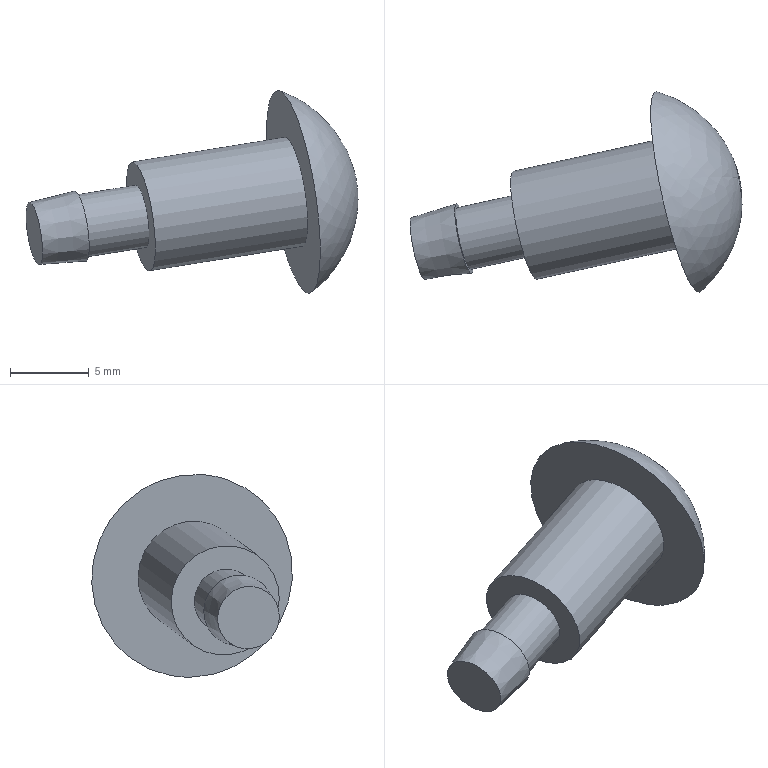Component | NX | 2_13 | 1 solid | 8 faces | box 21.02 x 12.71 x 12.84 mm | volume 772 mm3 | plane 4 | cylinder 2 | spline 1 | cone 1 | commonest cylinder face diameters 7 x1 4 x1
STEP:
#1=CARTESIAN_POINT('',(0.,0.,0.));
#2=DIRECTION('',(0.,0.,1.));
#3=DIRECTION('',(1.,0.,0.));
#4=AXIS2_PLACEMENT_3D('',#1,#2,#3);
#5=CARTESIAN_POINT('',(138.921,125.393,-187.423));
#6=VERTEX_POINT('',#5);
#7=CARTESIAN_POINT('',(139.276,125.209,-189.382));
#8=DIRECTION('',(0.9653,0.21,0.1554));
#9=DIRECTION('',(-0.1779,0.09244,0.9797));
#10=AXIS2_PLACEMENT_3D('',#7,#8,#9);
#11=CIRCLE('',#10,2.);
#12=CARTESIAN_POINT('',(139.632,125.024,-191.342));
#13=DIRECTION('',(-0.9653,-0.21,-0.1554));
#14=DIRECTION('',(0.1779,-0.09244,-0.9797));
#15=AXIS2_PLACEMENT_3D('',#12,#13,#14);
#16=PLANE('',#15);
#17=CARTESIAN_POINT('',(-4.,0.));
#18=CARTESIAN_POINT('',(-4.,3.464));
#19=CARTESIAN_POINT('',(-1.,1.732));
#20=CARTESIAN_POINT('',(2.,0.));
#21=CARTESIAN_POINT('',(-1.,-1.732));
#22=CARTESIAN_POINT('',(-4.,-3.464));
#23=CARTESIAN_POINT('',(-4.,0.));
#24=(BOUNDED_CURVE()B_SPLINE_CURVE(2,(#17,#18,#19,#20,#21,#22,#23),.UNSPECIFIED.,.T.,.F.)B_SPLINE_CURVE_WITH_KNOTS((1,2,2,2,2,1),(-2.094,0.,2.094,4.189,6.283,8.378),.UNSPECIFIED.)CURVE()GEOMETRIC_REPRESENTATION_ITEM()RATIONAL_B_SPLINE_CURVE((1.,0.5,1.,0.5,1.,0.5,1.))REPRESENTATION_ITEM(''));
#25=(GEOMETRIC_REPRESENTATION_CONTEXT(2)PARAMETRIC_REPRESENTATION_CONTEXT()REPRESENTATION_CONTEXT('',''));
#26=DEFINITIONAL_REPRESENTATION('',(#24),#25);
#27=PCURVE('',#16,#26);
#28=CARTESIAN_POINT('',(142.172,125.839,-188.916));
#29=DIRECTION('',(0.9653,0.21,0.1554));
#30=DIRECTION('',(-0.1779,0.09244,0.9797));
#31=AXIS2_PLACEMENT_3D('',#28,#29,#30);
#32=CONICAL_SURFACE('',#31,2.25,0.08314);
#33=CARTESIAN_POINT('',(0.,-3.));
#34=DIRECTION('',(1.,0.));
#35=VECTOR('',#34,1.);
#36=LINE('',#33,#35);
#37=(GEOMETRIC_REPRESENTATION_CONTEXT(2)PARAMETRIC_REPRESENTATION_CONTEXT()REPRESENTATION_CONTEXT('',''));
#38=DEFINITIONAL_REPRESENTATION('',(#36),#37);
#39=PCURVE('',#32,#38);
#40=SURFACE_CURVE('',#11,(#27,#39),.PCURVE_S1.);
#41=EDGE_CURVE('',#6,#6,#40,.T.);
#42=ORIENTED_EDGE('',*,*,#41,.F.);
#43=EDGE_LOOP('',(#42));
#44=FACE_BOUND('',#43,.T.);
#45=ADVANCED_FACE('',(#44),#16,.T.);
#46=CARTESIAN_POINT('',(154.53,129.379,-180.372));
#47=VERTEX_POINT('',#46);
#48=CARTESIAN_POINT('',(155.686,128.779,-186.74));
#49=DIRECTION('',(0.9653,0.21,0.1554));
#50=DIRECTION('',(-0.1779,0.09244,0.9797));
#51=AXIS2_PLACEMENT_3D('',#48,#49,#50);
#52=CIRCLE('',#51,6.5);
#53=CARTESIAN_POINT('',(159.547,129.619,-186.118));
#54=CARTESIAN_POINT('',(159.547,129.619,-186.118));
#55=CARTESIAN_POINT('',(159.547,129.619,-186.118));
#56=CARTESIAN_POINT('',(159.547,129.619,-186.118));
#57=CARTESIAN_POINT('',(159.547,129.619,-186.118));
#58=CARTESIAN_POINT('',(159.547,129.619,-186.118));
#59=CARTESIAN_POINT('',(159.547,129.619,-186.118));
#60=CARTESIAN_POINT('',(159.,129.867,-183.379));
#61=CARTESIAN_POINT('',(160.073,124.409,-182.669));
#62=CARTESIAN_POINT('',(161.07,123.891,-188.163));
#63=CARTESIAN_POINT('',(159.997,129.349,-188.873));
#64=CARTESIAN_POINT('',(158.924,134.807,-189.582));
#65=CARTESIAN_POINT('',(157.927,135.325,-184.089));
#66=CARTESIAN_POINT('',(159.,129.867,-183.379));
#67=CARTESIAN_POINT('',(157.157,129.779,-181.268));
#68=CARTESIAN_POINT('',(159.144,119.673,-179.953));
#69=CARTESIAN_POINT('',(160.991,118.713,-190.126));
#70=CARTESIAN_POINT('',(159.003,128.82,-191.441));
#71=CARTESIAN_POINT('',(157.016,138.926,-192.755));
#72=CARTESIAN_POINT('',(155.169,139.886,-182.582));
#73=CARTESIAN_POINT('',(157.157,129.779,-181.268));
#74=CARTESIAN_POINT('',(154.53,129.379,-180.372));
#75=CARTESIAN_POINT('',(157.018,116.726,-178.726));
#76=CARTESIAN_POINT('',(159.33,115.525,-191.462));
#77=CARTESIAN_POINT('',(156.842,128.178,-193.108));
#78=CARTESIAN_POINT('',(154.354,140.831,-194.753));
#79=CARTESIAN_POINT('',(152.042,142.033,-182.017));
#80=CARTESIAN_POINT('',(154.53,129.379,-180.372));
#81=(BOUNDED_SURFACE()B_SPLINE_SURFACE(3,3,((#53,#54,#55,#56,#57,#58,#59),(#60,#61,#62,#63,#64,#65,#66),(#67,#68,#69,#70,#71,#72,#73),(#74,#75,#76,#77,#78,#79,#80)),.UNSPECIFIED.,.F.,.T.,.F.)B_SPLINE_SURFACE_WITH_KNOTS((4,4),(1,3,3,3,1),(0.,1.),(-0.5,0.,0.5,1.,1.5),.UNSPECIFIED.)GEOMETRIC_REPRESENTATION_ITEM()RATIONAL_B_SPLINE_SURFACE(((1.,0.3333,0.3333,1.,0.3333,0.3333,1.),(0.9073,0.3024,0.3024,0.9073,0.3024,0.3024,0.9073),(0.9073,0.3024,0.3024,0.9073,0.3024,0.3024,0.9073),(1.,0.3333,0.3333,1.,0.3333,0.3333,1.)))REPRESENTATION_ITEM('')SURFACE());
#82=CARTESIAN_POINT('',(1.,0.));
#83=CARTESIAN_POINT('',(1.,0.02352));
#84=CARTESIAN_POINT('',(1.,0.06491));
#85=CARTESIAN_POINT('',(1.,0.1146));
#86=CARTESIAN_POINT('',(1.,0.1575));
#87=CARTESIAN_POINT('',(1.,0.196));
#88=CARTESIAN_POINT('',(1.,0.2322));
#89=CARTESIAN_POINT('',(1.,0.2678));
#90=CARTESIAN_POINT('',(1.,0.304));
#91=CARTESIAN_POINT('',(1.,0.3425));
#92=CARTESIAN_POINT('',(1.,0.3856));
#93=CARTESIAN_POINT('',(1.,0.4343));
#94=CARTESIAN_POINT('',(1.,0.5));
#95=CARTESIAN_POINT('',(1.,0.5657));
#96=CARTESIAN_POINT('',(1.,0.6144));
#97=CARTESIAN_POINT('',(1.,0.6575));
#98=CARTESIAN_POINT('',(1.,0.696));
#99=CARTESIAN_POINT('',(1.,0.7322));
#100=CARTESIAN_POINT('',(1.,0.7678));
#101=CARTESIAN_POINT('',(1.,0.804));
#102=CARTESIAN_POINT('',(1.,0.8425));
#103=CARTESIAN_POINT('',(1.,0.8854));
#104=CARTESIAN_POINT('',(1.,0.9351));
#105=CARTESIAN_POINT('',(1.,0.9765));
#106=CARTESIAN_POINT('',(1.,1.));
#107=B_SPLINE_CURVE_WITH_KNOTS('',3,(#82,#83,#84,#85,#86,#87,#88,#89,#90,#91,#92,#93,#94,#95,#96,#97,#98,#99,#100,#101,#102,#103,#104,#105,#106),.UNSPECIFIED.,.F.,.F.,(4,1,1,1,1,1,1,1,1,1,1,1,1,1,1,1,1,1,1,1,1,1,4),(0.,0.2856,0.5712,0.8568,1.142,1.428,1.714,1.999,2.285,2.57,2.856,3.142,3.427,3.713,3.998,4.284,4.57,4.855,5.141,5.426,5.712,5.998,6.283),.QUASI_UNIFORM_KNOTS.);
#108=(GEOMETRIC_REPRESENTATION_CONTEXT(2)PARAMETRIC_REPRESENTATION_CONTEXT()REPRESENTATION_CONTEXT('',''));
#109=DEFINITIONAL_REPRESENTATION('',(#107),#108);
#110=PCURVE('',#81,#109);
#111=CARTESIAN_POINT('',(156.842,128.178,-193.108));
#112=DIRECTION('',(-0.9653,-0.21,-0.1554));
#113=DIRECTION('',(0.1779,-0.09244,-0.9797));
#114=AXIS2_PLACEMENT_3D('',#111,#112,#113);
#115=PLANE('',#114);
#116=CARTESIAN_POINT('',(-13.,-0.));
#117=CARTESIAN_POINT('',(-13.,11.258));
#118=CARTESIAN_POINT('',(-3.25,5.629));
#119=CARTESIAN_POINT('',(6.5,-0.));
#120=CARTESIAN_POINT('',(-3.25,-5.629));
#121=CARTESIAN_POINT('',(-13.,-11.258));
#122=CARTESIAN_POINT('',(-13.,-0.));
#123=(BOUNDED_CURVE()B_SPLINE_CURVE(2,(#116,#117,#118,#119,#120,#121,#122),.UNSPECIFIED.,.T.,.F.)B_SPLINE_CURVE_WITH_KNOTS((1,2,2,2,2,1),(-2.094,0.,2.094,4.189,6.283,8.378),.UNSPECIFIED.)CURVE()GEOMETRIC_REPRESENTATION_ITEM()RATIONAL_B_SPLINE_CURVE((1.,0.5,1.,0.5,1.,0.5,1.))REPRESENTATION_ITEM(''));
#124=(GEOMETRIC_REPRESENTATION_CONTEXT(2)PARAMETRIC_REPRESENTATION_CONTEXT()REPRESENTATION_CONTEXT('',''));
#125=DEFINITIONAL_REPRESENTATION('',(#123),#124);
#126=PCURVE('',#115,#125);
#127=SURFACE_CURVE('',#52,(#110,#126),.PCURVE_S1.);
#128=EDGE_CURVE('',#47,#47,#127,.T.);
#129=ORIENTED_EDGE('',*,*,#128,.T.);
#130=CARTESIAN_POINT('',(159.547,129.619,-186.118));
#131=VERTEX_POINT('',#130);
#132=CARTESIAN_POINT('',(159.547,129.619,-186.118));
#133=CARTESIAN_POINT('',(159.,129.867,-183.379));
#134=CARTESIAN_POINT('',(157.157,129.779,-181.268));
#135=CARTESIAN_POINT('',(154.53,129.379,-180.372));
#136=(BOUNDED_CURVE()B_SPLINE_CURVE(3,(#132,#133,#134,#135),.UNSPECIFIED.,.F.,.F.)B_SPLINE_CURVE_WITH_KNOTS((4,4),(0.,1.),.PIECEWISE_BEZIER_KNOTS.)CURVE()GEOMETRIC_REPRESENTATION_ITEM()RATIONAL_B_SPLINE_CURVE((1.,0.9073,0.9073,1.))REPRESENTATION_ITEM(''));
#137=CARTESIAN_POINT('',(0.,1.));
#138=DIRECTION('',(1.,0.));
#139=VECTOR('',#138,1.);
#140=LINE('',#137,#139);
#141=(GEOMETRIC_REPRESENTATION_CONTEXT(2)PARAMETRIC_REPRESENTATION_CONTEXT()REPRESENTATION_CONTEXT('',''));
#142=DEFINITIONAL_REPRESENTATION('',(#140),#141);
#143=PCURVE('',#81,#142);
#144=CARTESIAN_POINT('',(0.,0.));
#145=DIRECTION('',(1.,0.));
#146=VECTOR('',#145,1.);
#147=LINE('',#144,#146);
#148=(GEOMETRIC_REPRESENTATION_CONTEXT(2)PARAMETRIC_REPRESENTATION_CONTEXT()REPRESENTATION_CONTEXT('',''));
#149=DEFINITIONAL_REPRESENTATION('',(#147),#148);
#150=PCURVE('',#81,#149);
#151=SEAM_CURVE('',#136,(#143,#150),.PCURVE_S1.);
#152=EDGE_CURVE('',#131,#47,#151,.T.);
#153=ORIENTED_EDGE('',*,*,#152,.F.);
#154=ORIENTED_EDGE('',*,*,#152,.T.);
#155=EDGE_LOOP('',(#129,#153,#154));
#156=FACE_BOUND('',#155,.T.);
#157=ADVANCED_FACE('',(#156),#81,.T.);
#158=CARTESIAN_POINT('',(155.063,129.102,-183.311));
#159=VERTEX_POINT('',#158);
#160=CARTESIAN_POINT('',(155.686,128.779,-186.74));
#161=DIRECTION('',(0.9653,0.21,0.1554));
#162=DIRECTION('',(-0.1779,0.09244,0.9797));
#163=AXIS2_PLACEMENT_3D('',#160,#161,#162);
#164=CIRCLE('',#163,3.5);
#165=CARTESIAN_POINT('',(-10.,-0.));
#166=CARTESIAN_POINT('',(-10.,6.062));
#167=CARTESIAN_POINT('',(-4.75,3.031));
#168=CARTESIAN_POINT('',(0.5,-0.));
#169=CARTESIAN_POINT('',(-4.75,-3.031));
#170=CARTESIAN_POINT('',(-10.,-6.062));
#171=CARTESIAN_POINT('',(-10.,-0.));
#172=(BOUNDED_CURVE()B_SPLINE_CURVE(2,(#165,#166,#167,#168,#169,#170,#171),.UNSPECIFIED.,.T.,.F.)B_SPLINE_CURVE_WITH_KNOTS((1,2,2,2,2,1),(-2.094,0.,2.094,4.189,6.283,8.378),.UNSPECIFIED.)CURVE()GEOMETRIC_REPRESENTATION_ITEM()RATIONAL_B_SPLINE_CURVE((1.,0.5,1.,0.5,1.,0.5,1.))REPRESENTATION_ITEM(''));
#173=(GEOMETRIC_REPRESENTATION_CONTEXT(2)PARAMETRIC_REPRESENTATION_CONTEXT()REPRESENTATION_CONTEXT('',''));
#174=DEFINITIONAL_REPRESENTATION('',(#172),#173);
#175=PCURVE('',#115,#174);
#176=CARTESIAN_POINT('',(148.929,127.309,-187.828));
#177=DIRECTION('',(0.9653,0.21,0.1554));
#178=DIRECTION('',(-0.1779,0.09244,0.9797));
#179=AXIS2_PLACEMENT_3D('',#176,#177,#178);
#180=CYLINDRICAL_SURFACE('',#179,3.5);
#181=CARTESIAN_POINT('',(0.,7.));
#182=DIRECTION('',(1.,0.));
#183=VECTOR('',#182,1.);
#184=LINE('',#181,#183);
#185=(GEOMETRIC_REPRESENTATION_CONTEXT(2)PARAMETRIC_REPRESENTATION_CONTEXT()REPRESENTATION_CONTEXT('',''));
#186=DEFINITIONAL_REPRESENTATION('',(#184),#185);
#187=PCURVE('',#180,#186);
#188=SURFACE_CURVE('',#164,(#175,#187),.PCURVE_S1.);
#189=EDGE_CURVE('',#159,#159,#188,.T.);
#190=ORIENTED_EDGE('',*,*,#189,.T.);
#191=EDGE_LOOP('',(#190));
#192=FACE_BOUND('',#191,.T.);
#193=ORIENTED_EDGE('',*,*,#128,.F.);
#194=EDGE_LOOP('',(#193));
#195=FACE_BOUND('',#194,.T.);
#196=ADVANCED_FACE('',(#192,#195),#115,.T.);
#197=CARTESIAN_POINT('',(145.411,127.002,-184.865));
#198=VERTEX_POINT('',#197);
#199=CARTESIAN_POINT('',(146.033,126.679,-188.294));
#200=DIRECTION('',(0.9653,0.21,0.1554));
#201=DIRECTION('',(-0.1779,0.09244,0.9797));
#202=AXIS2_PLACEMENT_3D('',#199,#200,#201);
#203=CIRCLE('',#202,3.5);
#204=CARTESIAN_POINT('',(0.,-3.));
#205=DIRECTION('',(1.,0.));
#206=VECTOR('',#205,1.);
#207=LINE('',#204,#206);
#208=(GEOMETRIC_REPRESENTATION_CONTEXT(2)PARAMETRIC_REPRESENTATION_CONTEXT()REPRESENTATION_CONTEXT('',''));
#209=DEFINITIONAL_REPRESENTATION('',(#207),#208);
#210=PCURVE('',#180,#209);
#211=CARTESIAN_POINT('',(146.656,126.355,-191.723));
#212=DIRECTION('',(-0.9653,-0.21,-0.1554));
#213=DIRECTION('',(0.1779,-0.09244,-0.9797));
#214=AXIS2_PLACEMENT_3D('',#211,#212,#213);
#215=PLANE('',#214);
#216=CARTESIAN_POINT('',(-7.,-0.));
#217=CARTESIAN_POINT('',(-7.,6.062));
#218=CARTESIAN_POINT('',(-1.75,3.031));
#219=CARTESIAN_POINT('',(3.5,-0.));
#220=CARTESIAN_POINT('',(-1.75,-3.031));
#221=CARTESIAN_POINT('',(-7.,-6.062));
#222=CARTESIAN_POINT('',(-7.,-0.));
#223=(BOUNDED_CURVE()B_SPLINE_CURVE(2,(#216,#217,#218,#219,#220,#221,#222),.UNSPECIFIED.,.T.,.F.)B_SPLINE_CURVE_WITH_KNOTS((1,2,2,2,2,1),(-2.094,0.,2.094,4.189,6.283,8.378),.UNSPECIFIED.)CURVE()GEOMETRIC_REPRESENTATION_ITEM()RATIONAL_B_SPLINE_CURVE((1.,0.5,1.,0.5,1.,0.5,1.))REPRESENTATION_ITEM(''));
#224=(GEOMETRIC_REPRESENTATION_CONTEXT(2)PARAMETRIC_REPRESENTATION_CONTEXT()REPRESENTATION_CONTEXT('',''));
#225=DEFINITIONAL_REPRESENTATION('',(#223),#224);
#226=PCURVE('',#215,#225);
#227=SURFACE_CURVE('',#203,(#210,#226),.PCURVE_S1.);
#228=EDGE_CURVE('',#198,#198,#227,.T.);
#229=ORIENTED_EDGE('',*,*,#228,.T.);
#230=CARTESIAN_POINT('',(145.411,127.002,-184.865));
#231=CARTESIAN_POINT('',(155.063,129.102,-183.311));
#232=B_SPLINE_CURVE_WITH_KNOTS('',1,(#230,#231),.UNSPECIFIED.,.F.,.F.,(2,2),(-3.,7.),.PIECEWISE_BEZIER_KNOTS.);
#233=CARTESIAN_POINT('',(6.283,0.));
#234=DIRECTION('',(0.,1.));
#235=VECTOR('',#234,1.);
#236=LINE('',#233,#235);
#237=(GEOMETRIC_REPRESENTATION_CONTEXT(2)PARAMETRIC_REPRESENTATION_CONTEXT()REPRESENTATION_CONTEXT('',''));
#238=DEFINITIONAL_REPRESENTATION('',(#236),#237);
#239=PCURVE('',#180,#238);
#240=CARTESIAN_POINT('',(0.,0.));
#241=DIRECTION('',(0.,1.));
#242=VECTOR('',#241,1.);
#243=LINE('',#240,#242);
#244=(GEOMETRIC_REPRESENTATION_CONTEXT(2)PARAMETRIC_REPRESENTATION_CONTEXT()REPRESENTATION_CONTEXT('',''));
#245=DEFINITIONAL_REPRESENTATION('',(#243),#244);
#246=PCURVE('',#180,#245);
#247=SEAM_CURVE('',#232,(#239,#246),.PCURVE_S1.);
#248=EDGE_CURVE('',#198,#159,#247,.T.);
#249=ORIENTED_EDGE('',*,*,#248,.T.);
#250=ORIENTED_EDGE('',*,*,#189,.F.);
#251=ORIENTED_EDGE('',*,*,#248,.F.);
#252=EDGE_LOOP('',(#229,#249,#250,#251));
#253=FACE_BOUND('',#252,.T.);
#254=ADVANCED_FACE('',(#253),#180,.T.);
#255=CARTESIAN_POINT('',(145.677,126.863,-186.335));
#256=VERTEX_POINT('',#255);
#257=CARTESIAN_POINT('',(146.033,126.679,-188.294));
#258=DIRECTION('',(0.9653,0.21,0.1554));
#259=DIRECTION('',(-0.1779,0.09244,0.9797));
#260=AXIS2_PLACEMENT_3D('',#257,#258,#259);
#261=CIRCLE('',#260,2.);
#262=CARTESIAN_POINT('',(-5.5,-0.));
#263=CARTESIAN_POINT('',(-5.5,3.464));
#264=CARTESIAN_POINT('',(-2.5,1.732));
#265=CARTESIAN_POINT('',(0.5,-0.));
#266=CARTESIAN_POINT('',(-2.5,-1.732));
#267=CARTESIAN_POINT('',(-5.5,-3.464));
#268=CARTESIAN_POINT('',(-5.5,-0.));
#269=(BOUNDED_CURVE()B_SPLINE_CURVE(2,(#262,#263,#264,#265,#266,#267,#268),.UNSPECIFIED.,.T.,.F.)B_SPLINE_CURVE_WITH_KNOTS((1,2,2,2,2,1),(-2.094,0.,2.094,4.189,6.283,8.378),.UNSPECIFIED.)CURVE()GEOMETRIC_REPRESENTATION_ITEM()RATIONAL_B_SPLINE_CURVE((1.,0.5,1.,0.5,1.,0.5,1.))REPRESENTATION_ITEM(''));
#270=(GEOMETRIC_REPRESENTATION_CONTEXT(2)PARAMETRIC_REPRESENTATION_CONTEXT()REPRESENTATION_CONTEXT('',''));
#271=DEFINITIONAL_REPRESENTATION('',(#269),#270);
#272=PCURVE('',#215,#271);
#273=CARTESIAN_POINT('',(148.929,127.309,-187.828));
#274=DIRECTION('',(0.9653,0.21,0.1554));
#275=DIRECTION('',(-0.1779,0.09244,0.9797));
#276=AXIS2_PLACEMENT_3D('',#273,#274,#275);
#277=CYLINDRICAL_SURFACE('',#276,2.);
#278=CARTESIAN_POINT('',(0.,-3.));
#279=DIRECTION('',(1.,0.));
#280=VECTOR('',#279,1.);
#281=LINE('',#278,#280);
#282=(GEOMETRIC_REPRESENTATION_CONTEXT(2)PARAMETRIC_REPRESENTATION_CONTEXT()REPRESENTATION_CONTEXT('',''));
#283=DEFINITIONAL_REPRESENTATION('',(#281),#282);
#284=PCURVE('',#277,#283);
#285=SURFACE_CURVE('',#261,(#272,#284),.PCURVE_S1.);
#286=EDGE_CURVE('',#256,#256,#285,.T.);
#287=ORIENTED_EDGE('',*,*,#286,.T.);
#288=EDGE_LOOP('',(#287));
#289=FACE_BOUND('',#288,.T.);
#290=ORIENTED_EDGE('',*,*,#228,.F.);
#291=EDGE_LOOP('',(#290));
#292=FACE_BOUND('',#291,.T.);
#293=ADVANCED_FACE('',(#289,#292),#215,.T.);
#294=CARTESIAN_POINT('',(141.816,126.023,-186.956));
#295=VERTEX_POINT('',#294);
#296=CARTESIAN_POINT('',(142.172,125.839,-188.916));
#297=DIRECTION('',(0.9653,0.21,0.1554));
#298=DIRECTION('',(-0.1779,0.09244,0.9797));
#299=AXIS2_PLACEMENT_3D('',#296,#297,#298);
#300=CIRCLE('',#299,2.);
#301=CARTESIAN_POINT('',(0.,-7.));
#302=DIRECTION('',(1.,0.));
#303=VECTOR('',#302,1.);
#304=LINE('',#301,#303);
#305=(GEOMETRIC_REPRESENTATION_CONTEXT(2)PARAMETRIC_REPRESENTATION_CONTEXT()REPRESENTATION_CONTEXT('',''));
#306=DEFINITIONAL_REPRESENTATION('',(#304),#305);
#307=PCURVE('',#277,#306);
#308=CARTESIAN_POINT('',(142.528,125.654,-190.875));
#309=DIRECTION('',(0.9653,0.21,0.1554));
#310=DIRECTION('',(-0.1779,0.09244,0.9797));
#311=AXIS2_PLACEMENT_3D('',#308,#309,#310);
#312=PLANE('',#311);
#313=CARTESIAN_POINT('',(2.,0.));
#314=DIRECTION('',(1.,-0.));
#315=AXIS2_PLACEMENT_2D('',#313,#314);
#316=CIRCLE('',#315,2.);
#317=(GEOMETRIC_REPRESENTATION_CONTEXT(2)PARAMETRIC_REPRESENTATION_CONTEXT()REPRESENTATION_CONTEXT('',''));
#318=DEFINITIONAL_REPRESENTATION('',(#316),#317);
#319=PCURVE('',#312,#318);
#320=SURFACE_CURVE('',#300,(#307,#319),.PCURVE_S1.);
#321=EDGE_CURVE('',#295,#295,#320,.T.);
#322=ORIENTED_EDGE('',*,*,#321,.T.);
#323=CARTESIAN_POINT('',(141.816,126.023,-186.956));
#324=CARTESIAN_POINT('',(145.677,126.863,-186.335));
#325=B_SPLINE_CURVE_WITH_KNOTS('',1,(#323,#324),.UNSPECIFIED.,.F.,.F.,(2,2),(-7.,-3.),.PIECEWISE_BEZIER_KNOTS.);
#326=CARTESIAN_POINT('',(6.283,0.));
#327=DIRECTION('',(0.,1.));
#328=VECTOR('',#327,1.);
#329=LINE('',#326,#328);
#330=(GEOMETRIC_REPRESENTATION_CONTEXT(2)PARAMETRIC_REPRESENTATION_CONTEXT()REPRESENTATION_CONTEXT('',''));
#331=DEFINITIONAL_REPRESENTATION('',(#329),#330);
#332=PCURVE('',#277,#331);
#333=CARTESIAN_POINT('',(0.,0.));
#334=DIRECTION('',(0.,1.));
#335=VECTOR('',#334,1.);
#336=LINE('',#333,#335);
#337=(GEOMETRIC_REPRESENTATION_CONTEXT(2)PARAMETRIC_REPRESENTATION_CONTEXT()REPRESENTATION_CONTEXT('',''));
#338=DEFINITIONAL_REPRESENTATION('',(#336),#337);
#339=PCURVE('',#277,#338);
#340=SEAM_CURVE('',#325,(#332,#339),.PCURVE_S1.);
#341=EDGE_CURVE('',#295,#256,#340,.T.);
#342=ORIENTED_EDGE('',*,*,#341,.T.);
#343=ORIENTED_EDGE('',*,*,#286,.F.);
#344=ORIENTED_EDGE('',*,*,#341,.F.);
#345=EDGE_LOOP('',(#322,#342,#343,#344));
#346=FACE_BOUND('',#345,.T.);
#347=ADVANCED_FACE('',(#346),#277,.T.);
#348=CARTESIAN_POINT('',(141.772,126.047,-186.712));
#349=VERTEX_POINT('',#348);
#350=CARTESIAN_POINT('',(142.172,125.839,-188.916));
#351=DIRECTION('',(0.9653,0.21,0.1554));
#352=DIRECTION('',(-0.1779,0.09244,0.9797));
#353=AXIS2_PLACEMENT_3D('',#350,#351,#352);
#354=CIRCLE('',#353,2.25);
#355=CARTESIAN_POINT('',(2.,0.));
#356=DIRECTION('',(1.,0.));
#357=AXIS2_PLACEMENT_2D('',#355,#356);
#358=CIRCLE('',#357,2.25);
#359=(GEOMETRIC_REPRESENTATION_CONTEXT(2)PARAMETRIC_REPRESENTATION_CONTEXT()REPRESENTATION_CONTEXT('',''));
#360=DEFINITIONAL_REPRESENTATION('',(#358),#359);
#361=PCURVE('',#312,#360);
#362=CARTESIAN_POINT('',(0.,0.));
#363=DIRECTION('',(1.,0.));
#364=VECTOR('',#363,1.);
#365=LINE('',#362,#364);
#366=(GEOMETRIC_REPRESENTATION_CONTEXT(2)PARAMETRIC_REPRESENTATION_CONTEXT()REPRESENTATION_CONTEXT('',''));
#367=DEFINITIONAL_REPRESENTATION('',(#365),#366);
#368=PCURVE('',#32,#367);
#369=SURFACE_CURVE('',#354,(#361,#368),.PCURVE_S1.);
#370=EDGE_CURVE('',#349,#349,#369,.T.);
#371=ORIENTED_EDGE('',*,*,#370,.T.);
#372=EDGE_LOOP('',(#371));
#373=FACE_BOUND('',#372,.T.);
#374=ORIENTED_EDGE('',*,*,#321,.F.);
#375=EDGE_LOOP('',(#374));
#376=FACE_BOUND('',#375,.T.);
#377=ADVANCED_FACE('',(#373,#376),#312,.T.);
#378=ORIENTED_EDGE('',*,*,#41,.T.);
#379=CARTESIAN_POINT('',(138.921,125.393,-187.423));
#380=CARTESIAN_POINT('',(141.772,126.047,-186.712));
#381=B_SPLINE_CURVE_WITH_KNOTS('',1,(#379,#380),.UNSPECIFIED.,.F.,.F.,(2,2),(-3.01,0.),.PIECEWISE_BEZIER_KNOTS.);
#382=CARTESIAN_POINT('',(6.283,0.));
#383=DIRECTION('',(0.,1.));
#384=VECTOR('',#383,1.);
#385=LINE('',#382,#384);
#386=(GEOMETRIC_REPRESENTATION_CONTEXT(2)PARAMETRIC_REPRESENTATION_CONTEXT()REPRESENTATION_CONTEXT('',''));
#387=DEFINITIONAL_REPRESENTATION('',(#385),#386);
#388=PCURVE('',#32,#387);
#389=CARTESIAN_POINT('',(0.,0.));
#390=DIRECTION('',(0.,1.));
#391=VECTOR('',#390,1.);
#392=LINE('',#389,#391);
#393=(GEOMETRIC_REPRESENTATION_CONTEXT(2)PARAMETRIC_REPRESENTATION_CONTEXT()REPRESENTATION_CONTEXT('',''));
#394=DEFINITIONAL_REPRESENTATION('',(#392),#393);
#395=PCURVE('',#32,#394);
#396=SEAM_CURVE('',#381,(#388,#395),.PCURVE_S1.);
#397=EDGE_CURVE('',#6,#349,#396,.T.);
#398=ORIENTED_EDGE('',*,*,#397,.T.);
#399=ORIENTED_EDGE('',*,*,#370,.F.);
#400=ORIENTED_EDGE('',*,*,#397,.F.);
#401=EDGE_LOOP('',(#378,#398,#399,#400));
#402=FACE_BOUND('',#401,.T.);
#403=ADVANCED_FACE('',(#402),#32,.T.);
#404=CLOSED_SHELL('',(#45,#157,#196,#254,#293,#347,#377,#403));
#405=MANIFOLD_SOLID_BREP('',#404);
#406=(LENGTH_UNIT()NAMED_UNIT(*)SI_UNIT(.MILLI.,.METRE.));
#407=UNCERTAINTY_MEASURE_WITH_UNIT(LENGTH_MEASURE(0.00001),#406,'','');
#408=(NAMED_UNIT(*)PLANE_ANGLE_UNIT()SI_UNIT($,.RADIAN.));
#409=(NAMED_UNIT(*)SI_UNIT($,.STERADIAN.)SOLID_ANGLE_UNIT());
#410=(GEOMETRIC_REPRESENTATION_CONTEXT(3)GLOBAL_UNCERTAINTY_ASSIGNED_CONTEXT((#407))GLOBAL_UNIT_ASSIGNED_CONTEXT((#406,#408,#409))REPRESENTATION_CONTEXT('',''));
#411=ADVANCED_BREP_SHAPE_REPRESENTATION('',(#4,#405),#410);